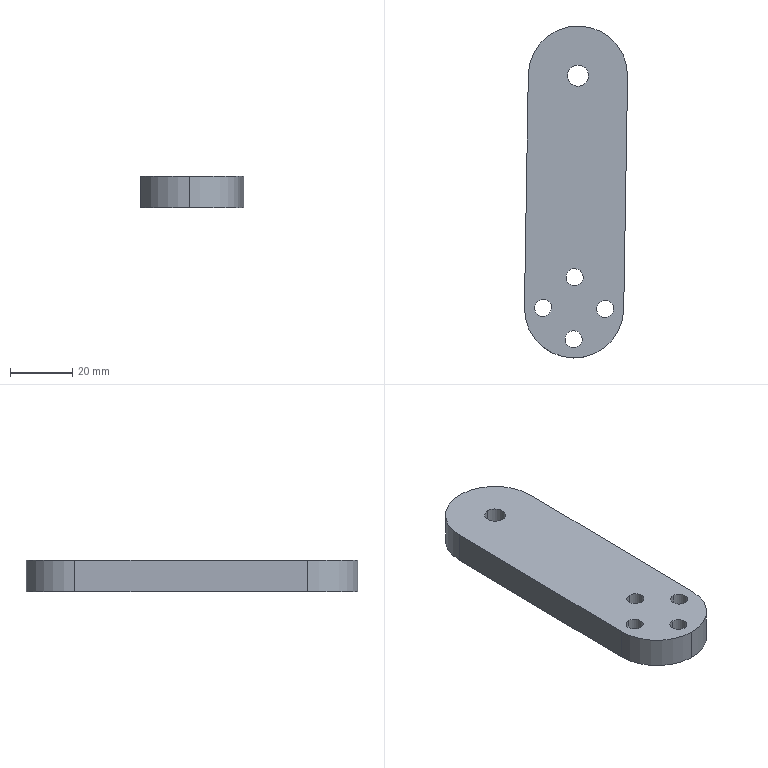Component | SolidWorks | 75-02-16StirringConnectingRod-1 | 1 solid | 29 faces | box 33.24 x 106.99 x 10 mm | volume 29480 mm3 | cylinder 21 | plane 8 | commonest cylinder face diameters 10 x8 5.5 x8 32 x3 6.8 x2 | material A3 Steel
build123d program:
from build123d import *

# Parameters (mm, degrees)
BOSS_EXTRUDE1_DEPTH                                = 5
HOLE_SIZE_ACCORDING_TO_TYPE_OF_HEXAGON_D           = 5.5
HOLE_SIZE_ACCORDING_TO_TYPE_OF_HEXAGON_CBORE_D     = 10
HOLE_SIZE_ACCORDING_TO_TYPE_OF_HEXAGON_CBORE_DEPTH = 5.7
M8_TAPPED_HOLE1_D                                  = 6.8


with BuildPart() as part:
    # Sketch1 → Boss-Extrude1 (new, symmetric)
    with BuildSketch(Plane.XY):
        with BuildLine():
            Line((-37.5, 16), (37.5, 16))
            ThreePointArc((37.5, 16), (53.5, 0), (37.5, -16))
            Line((37.5, -16), (-37.5, -16))
            ThreePointArc((-37.5, -16), (-53.5, 0), (-37.5, 16))
        make_face()
    extrude(amount=BOSS_EXTRUDE1_DEPTH, both=True)

    # Hole Size _according to_ Type of Hexagon (through all)
    with Locations(Plane(origin=(-37.5, 10, 5), x_dir=(1, 0, 0), z_dir=(0, 0, 1))):
        with Locations((0, 0), (10, -10), (-10, -10), (0, -20)):
            CounterBoreHole(HOLE_SIZE_ACCORDING_TO_TYPE_OF_HEXAGON_D / 2, HOLE_SIZE_ACCORDING_TO_TYPE_OF_HEXAGON_CBORE_D / 2, HOLE_SIZE_ACCORDING_TO_TYPE_OF_HEXAGON_CBORE_DEPTH)

    # M8 Tapped Hole1 (through all)
    with Locations(Plane(origin=(37.5, 0, 5), x_dir=(1, 0, 0), z_dir=(0, 0, 1))):
        with Locations((0, 0)):
            Hole(M8_TAPPED_HOLE1_D / 2)


solid = part.part

# Placed as in the assembly
solid = solid.moved(Location((-17.178, 49.362, 71.25), (-180, 0, -89.049)))
STEP:
#1=COLOUR_RGB('',0.7922,0.8196,0.9333);
#2=FILL_AREA_STYLE_COLOUR('',#1);
#3=FILL_AREA_STYLE('',(#2));
#4=SURFACE_STYLE_FILL_AREA(#3);
#5=SURFACE_SIDE_STYLE('',(#4));
#6=SURFACE_STYLE_USAGE(.BOTH.,#5);
#7=PRESENTATION_STYLE_ASSIGNMENT((#6));
#8=CARTESIAN_POINT('',(-0.654,3.286,3.002));
#9=VERTEX_POINT('',#8);
#10=CARTESIAN_POINT('',(-0.6496,3.553,3.002));
#11=VERTEX_POINT('',#10);
#12=CARTESIAN_POINT('',(-0.6518,3.42,3.002));
#13=DIRECTION('',(0.,0.,-1.));
#14=DIRECTION('',(0.0166,0.9999,0.));
#15=AXIS2_PLACEMENT_3D('',#12,#13,#14);
#16=CIRCLE('',#15,0.1339);
#17=EDGE_CURVE('',#9,#11,#16,.T.);
#18=ORIENTED_EDGE('',*,*,#17,.F.);
#19=CARTESIAN_POINT('',(-0.654,3.286,2.608));
#20=VERTEX_POINT('',#19);
#21=CARTESIAN_POINT('',(-0.654,3.286,2.608));
#22=DIRECTION('',(0.,0.,-1.));
#23=VECTOR('',#22,39.37);
#24=LINE('',#21,#23);
#25=EDGE_CURVE('',#9,#20,#24,.T.);
#26=ORIENTED_EDGE('',*,*,#25,.T.);
#27=CARTESIAN_POINT('',(-0.6496,3.553,2.608));
#28=VERTEX_POINT('',#27);
#29=CARTESIAN_POINT('',(-0.6518,3.42,2.608));
#30=DIRECTION('',(0.,0.,-1.));
#31=DIRECTION('',(0.0166,0.9999,0.));
#32=AXIS2_PLACEMENT_3D('',#29,#30,#31);
#33=CIRCLE('',#32,0.1339);
#34=EDGE_CURVE('',#20,#28,#33,.T.);
#35=ORIENTED_EDGE('',*,*,#34,.T.);
#36=CARTESIAN_POINT('',(-0.6496,3.553,2.608));
#37=DIRECTION('',(0.,0.,-1.));
#38=VECTOR('',#37,39.37);
#39=LINE('',#36,#38);
#40=EDGE_CURVE('',#11,#28,#39,.T.);
#41=ORIENTED_EDGE('',*,*,#40,.F.);
#42=EDGE_LOOP('',(#18,#26,#35,#41));
#43=FACE_OUTER_BOUND('',#42,.T.);
#44=CARTESIAN_POINT('',(-0.6518,3.42,2.608));
#45=DIRECTION('',(0.,0.,-1.));
#46=DIRECTION('',(0.0166,0.9999,0.));
#47=AXIS2_PLACEMENT_3D('',#44,#45,#46);
#48=CYLINDRICAL_SURFACE('',#47,0.1339);
#49=ADVANCED_FACE('',(#43),#48,.F.);
#50=CARTESIAN_POINT('',(-0.3104,0.2638,2.833));
#51=VERTEX_POINT('',#50);
#52=CARTESIAN_POINT('',(-0.3039,0.6575,2.833));
#53=VERTEX_POINT('',#52);
#54=CARTESIAN_POINT('',(-0.3072,0.4607,2.833));
#55=DIRECTION('',(0.,0.,-1.));
#56=DIRECTION('',(0.0166,0.9999,0.));
#57=AXIS2_PLACEMENT_3D('',#54,#55,#56);
#58=CIRCLE('',#57,0.1969);
#59=EDGE_CURVE('',#51,#53,#58,.T.);
#60=ORIENTED_EDGE('',*,*,#59,.F.);
#61=CARTESIAN_POINT('',(-0.3104,0.2638,2.608));
#62=VERTEX_POINT('',#61);
#63=CARTESIAN_POINT('',(-0.3104,0.2638,2.608));
#64=DIRECTION('',(0.,0.,-1.));
#65=VECTOR('',#64,39.37);
#66=LINE('',#63,#65);
#67=EDGE_CURVE('',#51,#62,#66,.T.);
#68=ORIENTED_EDGE('',*,*,#67,.T.);
#69=CARTESIAN_POINT('',(-0.3039,0.6575,2.608));
#70=VERTEX_POINT('',#69);
#71=CARTESIAN_POINT('',(-0.3072,0.4607,2.608));
#72=DIRECTION('',(0.,0.,-1.));
#73=DIRECTION('',(0.0166,0.9999,0.));
#74=AXIS2_PLACEMENT_3D('',#71,#72,#73);
#75=CIRCLE('',#74,0.1969);
#76=EDGE_CURVE('',#62,#70,#75,.T.);
#77=ORIENTED_EDGE('',*,*,#76,.T.);
#78=CARTESIAN_POINT('',(-0.3039,0.6575,2.608));
#79=DIRECTION('',(0.,0.,-1.));
#80=VECTOR('',#79,39.37);
#81=LINE('',#78,#80);
#82=EDGE_CURVE('',#53,#70,#81,.T.);
#83=ORIENTED_EDGE('',*,*,#82,.F.);
#84=EDGE_LOOP('',(#60,#68,#77,#83));
#85=FACE_OUTER_BOUND('',#84,.T.);
#86=CARTESIAN_POINT('',(-0.3072,0.4607,2.608));
#87=DIRECTION('',(0.,0.,-1.));
#88=DIRECTION('',(0.0166,0.9999,0.));
#89=AXIS2_PLACEMENT_3D('',#86,#87,#88);
#90=CYLINDRICAL_SURFACE('',#89,0.1969);
#91=ADVANCED_FACE('',(#85),#90,.F.);
#92=CARTESIAN_POINT('',(-0.309,0.3524,3.002));
#93=VERTEX_POINT('',#92);
#94=CARTESIAN_POINT('',(-0.3054,0.5689,3.002));
#95=VERTEX_POINT('',#94);
#96=CARTESIAN_POINT('',(-0.3072,0.4607,3.002));
#97=DIRECTION('',(0.,0.,-1.));
#98=DIRECTION('',(0.0166,0.9999,0.));
#99=AXIS2_PLACEMENT_3D('',#96,#97,#98);
#100=CIRCLE('',#99,0.1083);
#101=EDGE_CURVE('',#93,#95,#100,.T.);
#102=ORIENTED_EDGE('',*,*,#101,.F.);
#103=CARTESIAN_POINT('',(-0.309,0.3524,2.833));
#104=VERTEX_POINT('',#103);
#105=CARTESIAN_POINT('',(-0.309,0.3524,2.608));
#106=DIRECTION('',(0.,0.,-1.));
#107=VECTOR('',#106,39.37);
#108=LINE('',#105,#107);
#109=EDGE_CURVE('',#93,#104,#108,.T.);
#110=ORIENTED_EDGE('',*,*,#109,.T.);
#111=CARTESIAN_POINT('',(-0.3054,0.5689,2.833));
#112=VERTEX_POINT('',#111);
#113=CARTESIAN_POINT('',(-0.3072,0.4607,2.833));
#114=DIRECTION('',(0.,0.,-1.));
#115=DIRECTION('',(0.0166,0.9999,0.));
#116=AXIS2_PLACEMENT_3D('',#113,#114,#115);
#117=CIRCLE('',#116,0.1083);
#118=EDGE_CURVE('',#104,#112,#117,.T.);
#119=ORIENTED_EDGE('',*,*,#118,.T.);
#120=CARTESIAN_POINT('',(-0.3054,0.5689,2.608));
#121=DIRECTION('',(0.,0.,-1.));
#122=VECTOR('',#121,39.37);
#123=LINE('',#120,#122);
#124=EDGE_CURVE('',#95,#112,#123,.T.);
#125=ORIENTED_EDGE('',*,*,#124,.F.);
#126=EDGE_LOOP('',(#102,#110,#119,#125));
#127=FACE_OUTER_BOUND('',#126,.T.);
#128=CARTESIAN_POINT('',(-0.3072,0.4607,2.608));
#129=DIRECTION('',(0.,0.,-1.));
#130=DIRECTION('',(0.0166,0.9999,0.));
#131=AXIS2_PLACEMENT_3D('',#128,#129,#130);
#132=CYLINDRICAL_SURFACE('',#131,0.1083);
#133=ADVANCED_FACE('',(#127),#132,.F.);
#134=CARTESIAN_POINT('',(-0.6975,0.664,2.833));
#135=VERTEX_POINT('',#134);
#136=CARTESIAN_POINT('',(-0.691,1.058,2.833));
#137=VERTEX_POINT('',#136);
#138=CARTESIAN_POINT('',(-0.6943,0.8608,2.833));
#139=DIRECTION('',(0.,0.,-1.));
#140=DIRECTION('',(0.0166,0.9999,0.));
#141=AXIS2_PLACEMENT_3D('',#138,#139,#140);
#142=CIRCLE('',#141,0.1969);
#143=EDGE_CURVE('',#135,#137,#142,.T.);
#144=ORIENTED_EDGE('',*,*,#143,.F.);
#145=CARTESIAN_POINT('',(-0.6975,0.664,2.608));
#146=VERTEX_POINT('',#145);
#147=CARTESIAN_POINT('',(-0.6975,0.664,2.608));
#148=DIRECTION('',(0.,0.,-1.));
#149=VECTOR('',#148,39.37);
#150=LINE('',#147,#149);
#151=EDGE_CURVE('',#135,#146,#150,.T.);
#152=ORIENTED_EDGE('',*,*,#151,.T.);
#153=CARTESIAN_POINT('',(-0.691,1.058,2.608));
#154=VERTEX_POINT('',#153);
#155=CARTESIAN_POINT('',(-0.6943,0.8608,2.608));
#156=DIRECTION('',(0.,0.,-1.));
#157=DIRECTION('',(0.0166,0.9999,0.));
#158=AXIS2_PLACEMENT_3D('',#155,#156,#157);
#159=CIRCLE('',#158,0.1969);
#160=EDGE_CURVE('',#146,#154,#159,.T.);
#161=ORIENTED_EDGE('',*,*,#160,.T.);
#162=CARTESIAN_POINT('',(-0.691,1.058,2.608));
#163=DIRECTION('',(0.,0.,-1.));
#164=VECTOR('',#163,39.37);
#165=LINE('',#162,#164);
#166=EDGE_CURVE('',#137,#154,#165,.T.);
#167=ORIENTED_EDGE('',*,*,#166,.F.);
#168=EDGE_LOOP('',(#144,#152,#161,#167));
#169=FACE_OUTER_BOUND('',#168,.T.);
#170=CARTESIAN_POINT('',(-0.6943,0.8608,2.608));
#171=DIRECTION('',(0.,0.,-1.));
#172=DIRECTION('',(0.0166,0.9999,0.));
#173=AXIS2_PLACEMENT_3D('',#170,#171,#172);
#174=CYLINDRICAL_SURFACE('',#173,0.1969);
#175=ADVANCED_FACE('',(#169),#174,.F.);
#176=CARTESIAN_POINT('',(-0.6961,0.7526,3.002));
#177=VERTEX_POINT('',#176);
#178=CARTESIAN_POINT('',(-0.6925,0.9691,3.002));
#179=VERTEX_POINT('',#178);
#180=CARTESIAN_POINT('',(-0.6943,0.8608,3.002));
#181=DIRECTION('',(0.,0.,-1.));
#182=DIRECTION('',(0.0166,0.9999,0.));
#183=AXIS2_PLACEMENT_3D('',#180,#181,#182);
#184=CIRCLE('',#183,0.1083);
#185=EDGE_CURVE('',#177,#179,#184,.T.);
#186=ORIENTED_EDGE('',*,*,#185,.F.);
#187=CARTESIAN_POINT('',(-0.6961,0.7526,2.833));
#188=VERTEX_POINT('',#187);
#189=CARTESIAN_POINT('',(-0.6961,0.7526,2.608));
#190=DIRECTION('',(0.,0.,-1.));
#191=VECTOR('',#190,39.37);
#192=LINE('',#189,#191);
#193=EDGE_CURVE('',#177,#188,#192,.T.);
#194=ORIENTED_EDGE('',*,*,#193,.T.);
#195=CARTESIAN_POINT('',(-0.6925,0.9691,2.833));
#196=VERTEX_POINT('',#195);
#197=CARTESIAN_POINT('',(-0.6943,0.8608,2.833));
#198=DIRECTION('',(0.,0.,-1.));
#199=DIRECTION('',(0.0166,0.9999,0.));
#200=AXIS2_PLACEMENT_3D('',#197,#198,#199);
#201=CIRCLE('',#200,0.1083);
#202=EDGE_CURVE('',#188,#196,#201,.T.);
#203=ORIENTED_EDGE('',*,*,#202,.T.);
#204=CARTESIAN_POINT('',(-0.6925,0.9691,2.608));
#205=DIRECTION('',(0.,0.,-1.));
#206=VECTOR('',#205,39.37);
#207=LINE('',#204,#206);
#208=EDGE_CURVE('',#179,#196,#207,.T.);
#209=ORIENTED_EDGE('',*,*,#208,.F.);
#210=EDGE_LOOP('',(#186,#194,#203,#209));
#211=FACE_OUTER_BOUND('',#210,.T.);
#212=CARTESIAN_POINT('',(-0.6943,0.8608,2.608));
#213=DIRECTION('',(0.,0.,-1.));
#214=DIRECTION('',(0.0166,0.9999,0.));
#215=AXIS2_PLACEMENT_3D('',#212,#213,#214);
#216=CYLINDRICAL_SURFACE('',#215,0.1083);
#217=ADVANCED_FACE('',(#211),#216,.F.);
#218=CARTESIAN_POINT('',(-0.7106,-0.1233,2.833));
#219=VERTEX_POINT('',#218);
#220=CARTESIAN_POINT('',(-0.7041,0.2704,2.833));
#221=VERTEX_POINT('',#220);
#222=CARTESIAN_POINT('',(-0.7073,0.07355,2.833));
#223=DIRECTION('',(0.,0.,-1.));
#224=DIRECTION('',(0.0166,0.9999,0.));
#225=AXIS2_PLACEMENT_3D('',#222,#223,#224);
#226=CIRCLE('',#225,0.1969);
#227=EDGE_CURVE('',#219,#221,#226,.T.);
#228=ORIENTED_EDGE('',*,*,#227,.F.);
#229=CARTESIAN_POINT('',(-0.7106,-0.1233,2.608));
#230=VERTEX_POINT('',#229);
#231=CARTESIAN_POINT('',(-0.7106,-0.1233,2.608));
#232=DIRECTION('',(0.,0.,-1.));
#233=VECTOR('',#232,39.37);
#234=LINE('',#231,#233);
#235=EDGE_CURVE('',#219,#230,#234,.T.);
#236=ORIENTED_EDGE('',*,*,#235,.T.);
#237=CARTESIAN_POINT('',(-0.7041,0.2704,2.608));
#238=VERTEX_POINT('',#237);
#239=CARTESIAN_POINT('',(-0.7073,0.07355,2.608));
#240=DIRECTION('',(0.,0.,-1.));
#241=DIRECTION('',(0.0166,0.9999,0.));
#242=AXIS2_PLACEMENT_3D('',#239,#240,#241);
#243=CIRCLE('',#242,0.1969);
#244=EDGE_CURVE('',#230,#238,#243,.T.);
#245=ORIENTED_EDGE('',*,*,#244,.T.);
#246=CARTESIAN_POINT('',(-0.7041,0.2704,2.608));
#247=DIRECTION('',(0.,0.,-1.));
#248=VECTOR('',#247,39.37);
#249=LINE('',#246,#248);
#250=EDGE_CURVE('',#221,#238,#249,.T.);
#251=ORIENTED_EDGE('',*,*,#250,.F.);
#252=EDGE_LOOP('',(#228,#236,#245,#251));
#253=FACE_OUTER_BOUND('',#252,.T.);
#254=CARTESIAN_POINT('',(-0.7073,0.07355,2.608));
#255=DIRECTION('',(0.,0.,-1.));
#256=DIRECTION('',(0.0166,0.9999,0.));
#257=AXIS2_PLACEMENT_3D('',#254,#255,#256);
#258=CYLINDRICAL_SURFACE('',#257,0.1969);
#259=ADVANCED_FACE('',(#253),#258,.F.);
#260=CARTESIAN_POINT('',(-0.7091,-0.0347,3.002));
#261=VERTEX_POINT('',#260);
#262=CARTESIAN_POINT('',(-0.7055,0.1818,3.002));
#263=VERTEX_POINT('',#262);
#264=CARTESIAN_POINT('',(-0.7073,0.07355,3.002));
#265=DIRECTION('',(0.,0.,-1.));
#266=DIRECTION('',(0.0166,0.9999,0.));
#267=AXIS2_PLACEMENT_3D('',#264,#265,#266);
#268=CIRCLE('',#267,0.1083);
#269=EDGE_CURVE('',#261,#263,#268,.T.);
#270=ORIENTED_EDGE('',*,*,#269,.F.);
#271=CARTESIAN_POINT('',(-0.7091,-0.0347,2.833));
#272=VERTEX_POINT('',#271);
#273=CARTESIAN_POINT('',(-0.7091,-0.0347,2.608));
#274=DIRECTION('',(0.,0.,-1.));
#275=VECTOR('',#274,39.37);
#276=LINE('',#273,#275);
#277=EDGE_CURVE('',#261,#272,#276,.T.);
#278=ORIENTED_EDGE('',*,*,#277,.T.);
#279=CARTESIAN_POINT('',(-0.7055,0.1818,2.833));
#280=VERTEX_POINT('',#279);
#281=CARTESIAN_POINT('',(-0.7073,0.07355,2.833));
#282=DIRECTION('',(0.,0.,-1.));
#283=DIRECTION('',(0.0166,0.9999,0.));
#284=AXIS2_PLACEMENT_3D('',#281,#282,#283);
#285=CIRCLE('',#284,0.1083);
#286=EDGE_CURVE('',#272,#280,#285,.T.);
#287=ORIENTED_EDGE('',*,*,#286,.T.);
#288=CARTESIAN_POINT('',(-0.7055,0.1818,2.608));
#289=DIRECTION('',(0.,0.,-1.));
#290=VECTOR('',#289,39.37);
#291=LINE('',#288,#290);
#292=EDGE_CURVE('',#263,#280,#291,.T.);
#293=ORIENTED_EDGE('',*,*,#292,.F.);
#294=EDGE_LOOP('',(#270,#278,#287,#293));
#295=FACE_OUTER_BOUND('',#294,.T.);
#296=CARTESIAN_POINT('',(-0.7073,0.07355,2.608));
#297=DIRECTION('',(0.,0.,-1.));
#298=DIRECTION('',(0.0166,0.9999,0.));
#299=AXIS2_PLACEMENT_3D('',#296,#297,#298);
#300=CYLINDRICAL_SURFACE('',#299,0.1083);
#301=ADVANCED_FACE('',(#295),#300,.F.);
#302=CARTESIAN_POINT('',(-1.098,0.2769,2.833));
#303=VERTEX_POINT('',#302);
#304=CARTESIAN_POINT('',(-1.091,0.6706,2.833));
#305=VERTEX_POINT('',#304);
#306=CARTESIAN_POINT('',(-1.094,0.4737,2.833));
#307=DIRECTION('',(0.,0.,-1.));
#308=DIRECTION('',(0.0166,0.9999,0.));
#309=AXIS2_PLACEMENT_3D('',#306,#307,#308);
#310=CIRCLE('',#309,0.1969);
#311=EDGE_CURVE('',#303,#305,#310,.T.);
#312=ORIENTED_EDGE('',*,*,#311,.F.);
#313=CARTESIAN_POINT('',(-1.098,0.2769,2.608));
#314=VERTEX_POINT('',#313);
#315=CARTESIAN_POINT('',(-1.098,0.2769,2.608));
#316=DIRECTION('',(0.,0.,-1.));
#317=VECTOR('',#316,39.37);
#318=LINE('',#315,#317);
#319=EDGE_CURVE('',#303,#314,#318,.T.);
#320=ORIENTED_EDGE('',*,*,#319,.T.);
#321=CARTESIAN_POINT('',(-1.091,0.6706,2.608));
#322=VERTEX_POINT('',#321);
#323=CARTESIAN_POINT('',(-1.094,0.4737,2.608));
#324=DIRECTION('',(0.,0.,-1.));
#325=DIRECTION('',(0.0166,0.9999,0.));
#326=AXIS2_PLACEMENT_3D('',#323,#324,#325);
#327=CIRCLE('',#326,0.1969);
#328=EDGE_CURVE('',#314,#322,#327,.T.);
#329=ORIENTED_EDGE('',*,*,#328,.T.);
#330=CARTESIAN_POINT('',(-1.091,0.6706,2.608));
#331=DIRECTION('',(0.,0.,-1.));
#332=VECTOR('',#331,39.37);
#333=LINE('',#330,#332);
#334=EDGE_CURVE('',#305,#322,#333,.T.);
#335=ORIENTED_EDGE('',*,*,#334,.F.);
#336=EDGE_LOOP('',(#312,#320,#329,#335));
#337=FACE_OUTER_BOUND('',#336,.T.);
#338=CARTESIAN_POINT('',(-1.094,0.4737,2.608));
#339=DIRECTION('',(0.,0.,-1.));
#340=DIRECTION('',(0.0166,0.9999,0.));
#341=AXIS2_PLACEMENT_3D('',#338,#339,#340);
#342=CYLINDRICAL_SURFACE('',#341,0.1969);
#343=ADVANCED_FACE('',(#337),#342,.F.);
#344=CARTESIAN_POINT('',(-1.096,0.3655,3.002));
#345=VERTEX_POINT('',#344);
#346=CARTESIAN_POINT('',(-1.093,0.582,3.002));
#347=VERTEX_POINT('',#346);
#348=CARTESIAN_POINT('',(-1.094,0.4737,3.002));
#349=DIRECTION('',(0.,0.,-1.));
#350=DIRECTION('',(0.0166,0.9999,0.));
#351=AXIS2_PLACEMENT_3D('',#348,#349,#350);
#352=CIRCLE('',#351,0.1083);
#353=EDGE_CURVE('',#345,#347,#352,.T.);
#354=ORIENTED_EDGE('',*,*,#353,.F.);
#355=CARTESIAN_POINT('',(-1.096,0.3655,2.833));
#356=VERTEX_POINT('',#355);
#357=CARTESIAN_POINT('',(-1.096,0.3655,2.608));
#358=DIRECTION('',(0.,0.,-1.));
#359=VECTOR('',#358,39.37);
#360=LINE('',#357,#359);
#361=EDGE_CURVE('',#345,#356,#360,.T.);
#362=ORIENTED_EDGE('',*,*,#361,.T.);
#363=CARTESIAN_POINT('',(-1.093,0.582,2.833));
#364=VERTEX_POINT('',#363);
#365=CARTESIAN_POINT('',(-1.094,0.4737,2.833));
#366=DIRECTION('',(0.,0.,-1.));
#367=DIRECTION('',(0.0166,0.9999,0.));
#368=AXIS2_PLACEMENT_3D('',#365,#366,#367);
#369=CIRCLE('',#368,0.1083);
#370=EDGE_CURVE('',#356,#364,#369,.T.);
#371=ORIENTED_EDGE('',*,*,#370,.T.);
#372=CARTESIAN_POINT('',(-1.093,0.582,2.608));
#373=DIRECTION('',(0.,0.,-1.));
#374=VECTOR('',#373,39.37);
#375=LINE('',#372,#374);
#376=EDGE_CURVE('',#347,#364,#375,.T.);
#377=ORIENTED_EDGE('',*,*,#376,.F.);
#378=EDGE_LOOP('',(#354,#362,#371,#377));
#379=FACE_OUTER_BOUND('',#378,.T.);
#380=CARTESIAN_POINT('',(-1.094,0.4737,2.608));
#381=DIRECTION('',(0.,0.,-1.));
#382=DIRECTION('',(0.0166,0.9999,0.));
#383=AXIS2_PLACEMENT_3D('',#380,#381,#382);
#384=CYLINDRICAL_SURFACE('',#383,0.1083);
#385=ADVANCED_FACE('',(#379),#384,.F.);
#386=CARTESIAN_POINT('',(-0.7113,-0.1626,2.608));
#387=VERTEX_POINT('',#386);
#388=CARTESIAN_POINT('',(-1.331,0.4777,2.608));
#389=VERTEX_POINT('',#388);
#390=CARTESIAN_POINT('',(-0.7008,0.4672,2.608));
#391=DIRECTION('',(0.,0.,-1.));
#392=DIRECTION('',(0.0166,0.9999,0.));
#393=AXIS2_PLACEMENT_3D('',#390,#391,#392);
#394=CIRCLE('',#393,0.6299);
#395=EDGE_CURVE('',#387,#389,#394,.T.);
#396=ORIENTED_EDGE('',*,*,#395,.F.);
#397=CARTESIAN_POINT('',(-0.7113,-0.1626,3.002));
#398=VERTEX_POINT('',#397);
#399=CARTESIAN_POINT('',(-0.7113,-0.1626,2.608));
#400=DIRECTION('',(-0.,-0.,1.));
#401=VECTOR('',#400,39.37);
#402=LINE('',#399,#401);
#403=EDGE_CURVE('',#387,#398,#402,.T.);
#404=ORIENTED_EDGE('',*,*,#403,.T.);
#405=CARTESIAN_POINT('',(-1.331,0.4777,3.002));
#406=VERTEX_POINT('',#405);
#407=CARTESIAN_POINT('',(-0.7008,0.4672,3.002));
#408=DIRECTION('',(0.,0.,-1.));
#409=DIRECTION('',(0.0166,0.9999,0.));
#410=AXIS2_PLACEMENT_3D('',#407,#408,#409);
#411=CIRCLE('',#410,0.6299);
#412=EDGE_CURVE('',#398,#406,#411,.T.);
#413=ORIENTED_EDGE('',*,*,#412,.T.);
#414=CARTESIAN_POINT('',(-1.331,0.4777,2.608));
#415=DIRECTION('',(-0.,-0.,1.));
#416=VECTOR('',#415,39.37);
#417=LINE('',#414,#416);
#418=EDGE_CURVE('',#389,#406,#417,.T.);
#419=ORIENTED_EDGE('',*,*,#418,.F.);
#420=EDGE_LOOP('',(#396,#404,#413,#419));
#421=FACE_OUTER_BOUND('',#420,.T.);
#422=CARTESIAN_POINT('',(-0.7008,0.4672,2.608));
#423=DIRECTION('',(-0.,-0.,1.));
#424=DIRECTION('',(-0.0166,-0.9999,0.));
#425=AXIS2_PLACEMENT_3D('',#422,#423,#424);
#426=CYLINDRICAL_SURFACE('',#425,0.6299);
#427=ADVANCED_FACE('',(#421),#426,.T.);
#428=ORIENTED_EDGE('',*,*,#403,.F.);
#429=CARTESIAN_POINT('',(-0.07097,0.4567,2.608));
#430=VERTEX_POINT('',#429);
#431=CARTESIAN_POINT('',(-0.7008,0.4672,2.608));
#432=DIRECTION('',(0.,0.,-1.));
#433=DIRECTION('',(0.0166,0.9999,0.));
#434=AXIS2_PLACEMENT_3D('',#431,#432,#433);
#435=CIRCLE('',#434,0.6299);
#436=EDGE_CURVE('',#430,#387,#435,.T.);
#437=ORIENTED_EDGE('',*,*,#436,.F.);
#438=CARTESIAN_POINT('',(-0.07097,0.4567,3.002));
#439=VERTEX_POINT('',#438);
#440=CARTESIAN_POINT('',(-0.07097,0.4567,2.608));
#441=DIRECTION('',(-0.,-0.,1.));
#442=VECTOR('',#441,39.37);
#443=LINE('',#440,#442);
#444=EDGE_CURVE('',#430,#439,#443,.T.);
#445=ORIENTED_EDGE('',*,*,#444,.T.);
#446=CARTESIAN_POINT('',(-0.7008,0.4672,3.002));
#447=DIRECTION('',(0.,0.,-1.));
#448=DIRECTION('',(0.0166,0.9999,0.));
#449=AXIS2_PLACEMENT_3D('',#446,#447,#448);
#450=CIRCLE('',#449,0.6299);
#451=EDGE_CURVE('',#439,#398,#450,.T.);
#452=ORIENTED_EDGE('',*,*,#451,.T.);
#453=EDGE_LOOP('',(#428,#437,#445,#452));
#454=FACE_OUTER_BOUND('',#453,.T.);
#455=CARTESIAN_POINT('',(-0.7008,0.4672,2.608));
#456=DIRECTION('',(-0.,-0.,1.));
#457=DIRECTION('',(-0.0166,-0.9999,0.));
#458=AXIS2_PLACEMENT_3D('',#455,#456,#457);
#459=CYLINDRICAL_SURFACE('',#458,0.6299);
#460=ADVANCED_FACE('',(#454),#459,.T.);
#461=CARTESIAN_POINT('',(-1.282,3.43,3.002));
#462=VERTEX_POINT('',#461);
#463=CARTESIAN_POINT('',(-1.331,0.4777,3.002));
#464=DIRECTION('',(0.0166,0.9999,0.));
#465=VECTOR('',#464,39.37);
#466=LINE('',#463,#465);
#467=EDGE_CURVE('',#406,#462,#466,.T.);
#468=ORIENTED_EDGE('',*,*,#467,.T.);
#469=CARTESIAN_POINT('',(-1.282,3.43,2.608));
#470=VERTEX_POINT('',#469);
#471=CARTESIAN_POINT('',(-1.282,3.43,2.608));
#472=DIRECTION('',(-0.,-0.,1.));
#473=VECTOR('',#472,39.37);
#474=LINE('',#471,#473);
#475=EDGE_CURVE('',#470,#462,#474,.T.);
#476=ORIENTED_EDGE('',*,*,#475,.F.);
#477=CARTESIAN_POINT('',(-1.331,0.4777,2.608));
#478=DIRECTION('',(0.0166,0.9999,0.));
#479=VECTOR('',#478,39.37);
#480=LINE('',#477,#479);
#481=EDGE_CURVE('',#389,#470,#480,.T.);
#482=ORIENTED_EDGE('',*,*,#481,.F.);
#483=ORIENTED_EDGE('',*,*,#418,.T.);
#484=EDGE_LOOP('',(#468,#476,#482,#483));
#485=FACE_OUTER_BOUND('',#484,.T.);
#486=CARTESIAN_POINT('',(-1.331,0.4777,2.608));
#487=DIRECTION('',(0.9999,-0.0166,0.));
#488=DIRECTION('',(0.,0.,-1.));
#489=AXIS2_PLACEMENT_3D('',#486,#487,#488);
#490=PLANE('',#489);
#491=ADVANCED_FACE('',(#485),#490,.F.);
#492=CARTESIAN_POINT('',(-0.02196,3.409,3.002));
#493=VERTEX_POINT('',#492);
#494=CARTESIAN_POINT('',(-0.6518,3.42,3.002));
#495=DIRECTION('',(0.,0.,-1.));
#496=DIRECTION('',(0.0166,0.9999,0.));
#497=AXIS2_PLACEMENT_3D('',#494,#495,#496);
#498=CIRCLE('',#497,0.6299);
#499=EDGE_CURVE('',#462,#493,#498,.T.);
#500=ORIENTED_EDGE('',*,*,#499,.T.);
#501=CARTESIAN_POINT('',(-0.02196,3.409,2.608));
#502=VERTEX_POINT('',#501);
#503=CARTESIAN_POINT('',(-0.02196,3.409,2.608));
#504=DIRECTION('',(-0.,-0.,1.));
#505=VECTOR('',#504,39.37);
#506=LINE('',#503,#505);
#507=EDGE_CURVE('',#502,#493,#506,.T.);
#508=ORIENTED_EDGE('',*,*,#507,.F.);
#509=CARTESIAN_POINT('',(-0.6518,3.42,2.608));
#510=DIRECTION('',(0.,0.,-1.));
#511=DIRECTION('',(0.0166,0.9999,0.));
#512=AXIS2_PLACEMENT_3D('',#509,#510,#511);
#513=CIRCLE('',#512,0.6299);
#514=EDGE_CURVE('',#470,#502,#513,.T.);
#515=ORIENTED_EDGE('',*,*,#514,.F.);
#516=ORIENTED_EDGE('',*,*,#475,.T.);
#517=EDGE_LOOP('',(#500,#508,#515,#516));
#518=FACE_OUTER_BOUND('',#517,.T.);
#519=CARTESIAN_POINT('',(-0.6518,3.42,2.608));
#520=DIRECTION('',(-0.,-0.,1.));
#521=DIRECTION('',(-0.0166,-0.9999,0.));
#522=AXIS2_PLACEMENT_3D('',#519,#520,#521);
#523=CYLINDRICAL_SURFACE('',#522,0.6299);
#524=ADVANCED_FACE('',(#518),#523,.T.);
#525=CARTESIAN_POINT('',(-0.07097,0.4567,3.002));
#526=DIRECTION('',(-0.0166,-0.9999,-0.));
#527=VECTOR('',#526,39.37);
#528=LINE('',#525,#527);
#529=EDGE_CURVE('',#493,#439,#528,.T.);
#530=ORIENTED_EDGE('',*,*,#529,.T.);
#531=ORIENTED_EDGE('',*,*,#444,.F.);
#532=CARTESIAN_POINT('',(-0.07097,0.4567,2.608));
#533=DIRECTION('',(-0.0166,-0.9999,-0.));
#534=VECTOR('',#533,39.37);
#535=LINE('',#532,#534);
#536=EDGE_CURVE('',#502,#430,#535,.T.);
#537=ORIENTED_EDGE('',*,*,#536,.F.);
#538=ORIENTED_EDGE('',*,*,#507,.T.);
#539=EDGE_LOOP('',(#530,#531,#537,#538));
#540=FACE_OUTER_BOUND('',#539,.T.);
#541=CARTESIAN_POINT('',(-0.07097,0.4567,2.608));
#542=DIRECTION('',(-0.9999,0.0166,-0.));
#543=DIRECTION('',(-0.,-0.,1.));
#544=AXIS2_PLACEMENT_3D('',#541,#542,#543);
#545=PLANE('',#544);
#546=ADVANCED_FACE('',(#540),#545,.F.);
#547=CARTESIAN_POINT('',(-0.6518,3.42,2.608));
#548=DIRECTION('',(0.,0.,-1.));
#549=DIRECTION('',(0.0166,0.9999,0.));
#550=AXIS2_PLACEMENT_3D('',#547,#548,#549);
#551=CIRCLE('',#550,0.1339);
#552=EDGE_CURVE('',#28,#20,#551,.T.);
#553=ORIENTED_EDGE('',*,*,#552,.F.);
#554=ORIENTED_EDGE('',*,*,#34,.F.);
#555=EDGE_LOOP('',(#553,#554));
#556=FACE_BOUND('',#555,.T.);
#557=CARTESIAN_POINT('',(-0.3072,0.4607,2.608));
#558=DIRECTION('',(0.,0.,-1.));
#559=DIRECTION('',(0.0166,0.9999,0.));
#560=AXIS2_PLACEMENT_3D('',#557,#558,#559);
#561=CIRCLE('',#560,0.1969);
#562=EDGE_CURVE('',#70,#62,#561,.T.);
#563=ORIENTED_EDGE('',*,*,#562,.F.);
#564=ORIENTED_EDGE('',*,*,#76,.F.);
#565=EDGE_LOOP('',(#563,#564));
#566=FACE_BOUND('',#565,.T.);
#567=CARTESIAN_POINT('',(-0.6943,0.8608,2.608));
#568=DIRECTION('',(0.,0.,-1.));
#569=DIRECTION('',(0.0166,0.9999,0.));
#570=AXIS2_PLACEMENT_3D('',#567,#568,#569);
#571=CIRCLE('',#570,0.1969);
#572=EDGE_CURVE('',#154,#146,#571,.T.);
#573=ORIENTED_EDGE('',*,*,#572,.F.);
#574=ORIENTED_EDGE('',*,*,#160,.F.);
#575=EDGE_LOOP('',(#573,#574));
#576=FACE_BOUND('',#575,.T.);
#577=CARTESIAN_POINT('',(-0.7073,0.07355,2.608));
#578=DIRECTION('',(0.,0.,-1.));
#579=DIRECTION('',(0.0166,0.9999,0.));
#580=AXIS2_PLACEMENT_3D('',#577,#578,#579);
#581=CIRCLE('',#580,0.1969);
#582=EDGE_CURVE('',#238,#230,#581,.T.);
#583=ORIENTED_EDGE('',*,*,#582,.F.);
#584=ORIENTED_EDGE('',*,*,#244,.F.);
#585=EDGE_LOOP('',(#583,#584));
#586=FACE_BOUND('',#585,.T.);
#587=CARTESIAN_POINT('',(-1.094,0.4737,2.608));
#588=DIRECTION('',(0.,0.,-1.));
#589=DIRECTION('',(0.0166,0.9999,0.));
#590=AXIS2_PLACEMENT_3D('',#587,#588,#589);
#591=CIRCLE('',#590,0.1969);
#592=EDGE_CURVE('',#322,#314,#591,.T.);
#593=ORIENTED_EDGE('',*,*,#592,.F.);
#594=ORIENTED_EDGE('',*,*,#328,.F.);
#595=EDGE_LOOP('',(#593,#594));
#596=FACE_BOUND('',#595,.T.);
#597=ORIENTED_EDGE('',*,*,#436,.T.);
#598=ORIENTED_EDGE('',*,*,#395,.T.);
#599=ORIENTED_EDGE('',*,*,#481,.T.);
#600=ORIENTED_EDGE('',*,*,#514,.T.);
#601=ORIENTED_EDGE('',*,*,#536,.T.);
#602=EDGE_LOOP('',(#597,#598,#599,#600,#601));
#603=FACE_OUTER_BOUND('',#602,.T.);
#604=CARTESIAN_POINT('',(-0.7008,0.4672,2.608));
#605=DIRECTION('',(0.,0.,-1.));
#606=DIRECTION('',(0.0166,0.9999,0.));
#607=AXIS2_PLACEMENT_3D('',#604,#605,#606);
#608=PLANE('',#607);
#609=ADVANCED_FACE('',(#556,#566,#576,#586,#596,#603),#608,.T.);
#610=CARTESIAN_POINT('',(-0.6518,3.42,3.002));
#611=DIRECTION('',(0.,0.,-1.));
#612=DIRECTION('',(0.0166,0.9999,0.));
#613=AXIS2_PLACEMENT_3D('',#610,#611,#612);
#614=CIRCLE('',#613,0.1339);
#615=EDGE_CURVE('',#11,#9,#614,.T.);
#616=ORIENTED_EDGE('',*,*,#615,.T.);
#617=ORIENTED_EDGE('',*,*,#17,.T.);
#618=EDGE_LOOP('',(#616,#617));
#619=FACE_BOUND('',#618,.T.);
#620=CARTESIAN_POINT('',(-0.3072,0.4607,3.002));
#621=DIRECTION('',(0.,0.,-1.));
#622=DIRECTION('',(0.0166,0.9999,0.));
#623=AXIS2_PLACEMENT_3D('',#620,#621,#622);
#624=CIRCLE('',#623,0.1083);
#625=EDGE_CURVE('',#95,#93,#624,.T.);
#626=ORIENTED_EDGE('',*,*,#625,.T.);
#627=ORIENTED_EDGE('',*,*,#101,.T.);
#628=EDGE_LOOP('',(#626,#627));
#629=FACE_BOUND('',#628,.T.);
#630=CARTESIAN_POINT('',(-0.6943,0.8608,3.002));
#631=DIRECTION('',(0.,0.,-1.));
#632=DIRECTION('',(0.0166,0.9999,0.));
#633=AXIS2_PLACEMENT_3D('',#630,#631,#632);
#634=CIRCLE('',#633,0.1083);
#635=EDGE_CURVE('',#179,#177,#634,.T.);
#636=ORIENTED_EDGE('',*,*,#635,.T.);
#637=ORIENTED_EDGE('',*,*,#185,.T.);
#638=EDGE_LOOP('',(#636,#637));
#639=FACE_BOUND('',#638,.T.);
#640=CARTESIAN_POINT('',(-0.7073,0.07355,3.002));
#641=DIRECTION('',(0.,0.,-1.));
#642=DIRECTION('',(0.0166,0.9999,0.));
#643=AXIS2_PLACEMENT_3D('',#640,#641,#642);
#644=CIRCLE('',#643,0.1083);
#645=EDGE_CURVE('',#263,#261,#644,.T.);
#646=ORIENTED_EDGE('',*,*,#645,.T.);
#647=ORIENTED_EDGE('',*,*,#269,.T.);
#648=EDGE_LOOP('',(#646,#647));
#649=FACE_BOUND('',#648,.T.);
#650=CARTESIAN_POINT('',(-1.094,0.4737,3.002));
#651=DIRECTION('',(0.,0.,-1.));
#652=DIRECTION('',(0.0166,0.9999,0.));
#653=AXIS2_PLACEMENT_3D('',#650,#651,#652);
#654=CIRCLE('',#653,0.1083);
#655=EDGE_CURVE('',#347,#345,#654,.T.);
#656=ORIENTED_EDGE('',*,*,#655,.T.);
#657=ORIENTED_EDGE('',*,*,#353,.T.);
#658=EDGE_LOOP('',(#656,#657));
#659=FACE_BOUND('',#658,.T.);
#660=ORIENTED_EDGE('',*,*,#451,.F.);
#661=ORIENTED_EDGE('',*,*,#529,.F.);
#662=ORIENTED_EDGE('',*,*,#499,.F.);
#663=ORIENTED_EDGE('',*,*,#467,.F.);
#664=ORIENTED_EDGE('',*,*,#412,.F.);
#665=EDGE_LOOP('',(#660,#661,#662,#663,#664));
#666=FACE_OUTER_BOUND('',#665,.T.);
#667=CARTESIAN_POINT('',(-0.7008,0.4672,3.002));
#668=DIRECTION('',(0.,0.,-1.));
#669=DIRECTION('',(0.0166,0.9999,0.));
#670=AXIS2_PLACEMENT_3D('',#667,#668,#669);
#671=PLANE('',#670);
#672=ADVANCED_FACE('',(#619,#629,#639,#649,#659,#666),#671,.F.);
#673=ORIENTED_EDGE('',*,*,#361,.F.);
#674=ORIENTED_EDGE('',*,*,#655,.F.);
#675=ORIENTED_EDGE('',*,*,#376,.T.);
#676=CARTESIAN_POINT('',(-1.094,0.4737,2.833));
#677=DIRECTION('',(0.,0.,-1.));
#678=DIRECTION('',(0.0166,0.9999,0.));
#679=AXIS2_PLACEMENT_3D('',#676,#677,#678);
#680=CIRCLE('',#679,0.1083);
#681=EDGE_CURVE('',#364,#356,#680,.T.);
#682=ORIENTED_EDGE('',*,*,#681,.T.);
#683=EDGE_LOOP('',(#673,#674,#675,#682));
#684=FACE_OUTER_BOUND('',#683,.T.);
#685=CARTESIAN_POINT('',(-1.094,0.4737,2.608));
#686=DIRECTION('',(0.,0.,-1.));
#687=DIRECTION('',(0.0166,0.9999,0.));
#688=AXIS2_PLACEMENT_3D('',#685,#686,#687);
#689=CYLINDRICAL_SURFACE('',#688,0.1083);
#690=ADVANCED_FACE('',(#684),#689,.F.);
#691=ORIENTED_EDGE('',*,*,#681,.F.);
#692=ORIENTED_EDGE('',*,*,#370,.F.);
#693=EDGE_LOOP('',(#691,#692));
#694=FACE_BOUND('',#693,.T.);
#695=CARTESIAN_POINT('',(-1.094,0.4737,2.833));
#696=DIRECTION('',(0.,0.,-1.));
#697=DIRECTION('',(0.0166,0.9999,0.));
#698=AXIS2_PLACEMENT_3D('',#695,#696,#697);
#699=CIRCLE('',#698,0.1969);
#700=EDGE_CURVE('',#305,#303,#699,.T.);
#701=ORIENTED_EDGE('',*,*,#700,.T.);
#702=ORIENTED_EDGE('',*,*,#311,.T.);
#703=EDGE_LOOP('',(#701,#702));
#704=FACE_OUTER_BOUND('',#703,.T.);
#705=CARTESIAN_POINT('',(-1.093,0.582,2.833));
#706=DIRECTION('',(-0.,-0.,1.));
#707=DIRECTION('',(-0.0166,-0.9999,-0.));
#708=AXIS2_PLACEMENT_3D('',#705,#706,#707);
#709=PLANE('',#708);
#710=ADVANCED_FACE('',(#694,#704),#709,.F.);
#711=ORIENTED_EDGE('',*,*,#319,.F.);
#712=ORIENTED_EDGE('',*,*,#700,.F.);
#713=ORIENTED_EDGE('',*,*,#334,.T.);
#714=ORIENTED_EDGE('',*,*,#592,.T.);
#715=EDGE_LOOP('',(#711,#712,#713,#714));
#716=FACE_OUTER_BOUND('',#715,.T.);
#717=CARTESIAN_POINT('',(-1.094,0.4737,2.608));
#718=DIRECTION('',(0.,0.,-1.));
#719=DIRECTION('',(0.0166,0.9999,0.));
#720=AXIS2_PLACEMENT_3D('',#717,#718,#719);
#721=CYLINDRICAL_SURFACE('',#720,0.1969);
#722=ADVANCED_FACE('',(#716),#721,.F.);
#723=ORIENTED_EDGE('',*,*,#277,.F.);
#724=ORIENTED_EDGE('',*,*,#645,.F.);
#725=ORIENTED_EDGE('',*,*,#292,.T.);
#726=CARTESIAN_POINT('',(-0.7073,0.07355,2.833));
#727=DIRECTION('',(0.,0.,-1.));
#728=DIRECTION('',(0.0166,0.9999,0.));
#729=AXIS2_PLACEMENT_3D('',#726,#727,#728);
#730=CIRCLE('',#729,0.1083);
#731=EDGE_CURVE('',#280,#272,#730,.T.);
#732=ORIENTED_EDGE('',*,*,#731,.T.);
#733=EDGE_LOOP('',(#723,#724,#725,#732));
#734=FACE_OUTER_BOUND('',#733,.T.);
#735=CARTESIAN_POINT('',(-0.7073,0.07355,2.608));
#736=DIRECTION('',(0.,0.,-1.));
#737=DIRECTION('',(0.0166,0.9999,0.));
#738=AXIS2_PLACEMENT_3D('',#735,#736,#737);
#739=CYLINDRICAL_SURFACE('',#738,0.1083);
#740=ADVANCED_FACE('',(#734),#739,.F.);
#741=ORIENTED_EDGE('',*,*,#731,.F.);
#742=ORIENTED_EDGE('',*,*,#286,.F.);
#743=EDGE_LOOP('',(#741,#742));
#744=FACE_BOUND('',#743,.T.);
#745=CARTESIAN_POINT('',(-0.7073,0.07355,2.833));
#746=DIRECTION('',(0.,0.,-1.));
#747=DIRECTION('',(0.0166,0.9999,0.));
#748=AXIS2_PLACEMENT_3D('',#745,#746,#747);
#749=CIRCLE('',#748,0.1969);
#750=EDGE_CURVE('',#221,#219,#749,.T.);
#751=ORIENTED_EDGE('',*,*,#750,.T.);
#752=ORIENTED_EDGE('',*,*,#227,.T.);
#753=EDGE_LOOP('',(#751,#752));
#754=FACE_OUTER_BOUND('',#753,.T.);
#755=CARTESIAN_POINT('',(-0.7055,0.1818,2.833));
#756=DIRECTION('',(-0.,-0.,1.));
#757=DIRECTION('',(-0.0166,-0.9999,-0.));
#758=AXIS2_PLACEMENT_3D('',#755,#756,#757);
#759=PLANE('',#758);
#760=ADVANCED_FACE('',(#744,#754),#759,.F.);
#761=ORIENTED_EDGE('',*,*,#235,.F.);
#762=ORIENTED_EDGE('',*,*,#750,.F.);
#763=ORIENTED_EDGE('',*,*,#250,.T.);
#764=ORIENTED_EDGE('',*,*,#582,.T.);
#765=EDGE_LOOP('',(#761,#762,#763,#764));
#766=FACE_OUTER_BOUND('',#765,.T.);
#767=CARTESIAN_POINT('',(-0.7073,0.07355,2.608));
#768=DIRECTION('',(0.,0.,-1.));
#769=DIRECTION('',(0.0166,0.9999,0.));
#770=AXIS2_PLACEMENT_3D('',#767,#768,#769);
#771=CYLINDRICAL_SURFACE('',#770,0.1969);
#772=ADVANCED_FACE('',(#766),#771,.F.);
#773=ORIENTED_EDGE('',*,*,#193,.F.);
#774=ORIENTED_EDGE('',*,*,#635,.F.);
#775=ORIENTED_EDGE('',*,*,#208,.T.);
#776=CARTESIAN_POINT('',(-0.6943,0.8608,2.833));
#777=DIRECTION('',(0.,0.,-1.));
#778=DIRECTION('',(0.0166,0.9999,0.));
#779=AXIS2_PLACEMENT_3D('',#776,#777,#778);
#780=CIRCLE('',#779,0.1083);
#781=EDGE_CURVE('',#196,#188,#780,.T.);
#782=ORIENTED_EDGE('',*,*,#781,.T.);
#783=EDGE_LOOP('',(#773,#774,#775,#782));
#784=FACE_OUTER_BOUND('',#783,.T.);
#785=CARTESIAN_POINT('',(-0.6943,0.8608,2.608));
#786=DIRECTION('',(0.,0.,-1.));
#787=DIRECTION('',(0.0166,0.9999,0.));
#788=AXIS2_PLACEMENT_3D('',#785,#786,#787);
#789=CYLINDRICAL_SURFACE('',#788,0.1083);
#790=ADVANCED_FACE('',(#784),#789,.F.);
#791=ORIENTED_EDGE('',*,*,#781,.F.);
#792=ORIENTED_EDGE('',*,*,#202,.F.);
#793=EDGE_LOOP('',(#791,#792));
#794=FACE_BOUND('',#793,.T.);
#795=CARTESIAN_POINT('',(-0.6943,0.8608,2.833));
#796=DIRECTION('',(0.,0.,-1.));
#797=DIRECTION('',(0.0166,0.9999,0.));
#798=AXIS2_PLACEMENT_3D('',#795,#796,#797);
#799=CIRCLE('',#798,0.1969);
#800=EDGE_CURVE('',#137,#135,#799,.T.);
#801=ORIENTED_EDGE('',*,*,#800,.T.);
#802=ORIENTED_EDGE('',*,*,#143,.T.);
#803=EDGE_LOOP('',(#801,#802));
#804=FACE_OUTER_BOUND('',#803,.T.);
#805=CARTESIAN_POINT('',(-0.6925,0.9691,2.833));
#806=DIRECTION('',(-0.,-0.,1.));
#807=DIRECTION('',(-0.0166,-0.9999,-0.));
#808=AXIS2_PLACEMENT_3D('',#805,#806,#807);
#809=PLANE('',#808);
#810=ADVANCED_FACE('',(#794,#804),#809,.F.);
#811=ORIENTED_EDGE('',*,*,#151,.F.);
#812=ORIENTED_EDGE('',*,*,#800,.F.);
#813=ORIENTED_EDGE('',*,*,#166,.T.);
#814=ORIENTED_EDGE('',*,*,#572,.T.);
#815=EDGE_LOOP('',(#811,#812,#813,#814));
#816=FACE_OUTER_BOUND('',#815,.T.);
#817=CARTESIAN_POINT('',(-0.6943,0.8608,2.608));
#818=DIRECTION('',(0.,0.,-1.));
#819=DIRECTION('',(0.0166,0.9999,0.));
#820=AXIS2_PLACEMENT_3D('',#817,#818,#819);
#821=CYLINDRICAL_SURFACE('',#820,0.1969);
#822=ADVANCED_FACE('',(#816),#821,.F.);
#823=ORIENTED_EDGE('',*,*,#109,.F.);
#824=ORIENTED_EDGE('',*,*,#625,.F.);
#825=ORIENTED_EDGE('',*,*,#124,.T.);
#826=CARTESIAN_POINT('',(-0.3072,0.4607,2.833));
#827=DIRECTION('',(0.,0.,-1.));
#828=DIRECTION('',(0.0166,0.9999,0.));
#829=AXIS2_PLACEMENT_3D('',#826,#827,#828);
#830=CIRCLE('',#829,0.1083);
#831=EDGE_CURVE('',#112,#104,#830,.T.);
#832=ORIENTED_EDGE('',*,*,#831,.T.);
#833=EDGE_LOOP('',(#823,#824,#825,#832));
#834=FACE_OUTER_BOUND('',#833,.T.);
#835=CARTESIAN_POINT('',(-0.3072,0.4607,2.608));
#836=DIRECTION('',(0.,0.,-1.));
#837=DIRECTION('',(0.0166,0.9999,0.));
#838=AXIS2_PLACEMENT_3D('',#835,#836,#837);
#839=CYLINDRICAL_SURFACE('',#838,0.1083);
#840=ADVANCED_FACE('',(#834),#839,.F.);
#841=ORIENTED_EDGE('',*,*,#831,.F.);
#842=ORIENTED_EDGE('',*,*,#118,.F.);
#843=EDGE_LOOP('',(#841,#842));
#844=FACE_BOUND('',#843,.T.);
#845=CARTESIAN_POINT('',(-0.3072,0.4607,2.833));
#846=DIRECTION('',(0.,0.,-1.));
#847=DIRECTION('',(0.0166,0.9999,0.));
#848=AXIS2_PLACEMENT_3D('',#845,#846,#847);
#849=CIRCLE('',#848,0.1969);
#850=EDGE_CURVE('',#53,#51,#849,.T.);
#851=ORIENTED_EDGE('',*,*,#850,.T.);
#852=ORIENTED_EDGE('',*,*,#59,.T.);
#853=EDGE_LOOP('',(#851,#852));
#854=FACE_OUTER_BOUND('',#853,.T.);
#855=CARTESIAN_POINT('',(-0.3054,0.5689,2.833));
#856=DIRECTION('',(-0.,-0.,1.));
#857=DIRECTION('',(-0.0166,-0.9999,-0.));
#858=AXIS2_PLACEMENT_3D('',#855,#856,#857);
#859=PLANE('',#858);
#860=ADVANCED_FACE('',(#844,#854),#859,.F.);
#861=ORIENTED_EDGE('',*,*,#67,.F.);
#862=ORIENTED_EDGE('',*,*,#850,.F.);
#863=ORIENTED_EDGE('',*,*,#82,.T.);
#864=ORIENTED_EDGE('',*,*,#562,.T.);
#865=EDGE_LOOP('',(#861,#862,#863,#864));
#866=FACE_OUTER_BOUND('',#865,.T.);
#867=CARTESIAN_POINT('',(-0.3072,0.4607,2.608));
#868=DIRECTION('',(0.,0.,-1.));
#869=DIRECTION('',(0.0166,0.9999,0.));
#870=AXIS2_PLACEMENT_3D('',#867,#868,#869);
#871=CYLINDRICAL_SURFACE('',#870,0.1969);
#872=ADVANCED_FACE('',(#866),#871,.F.);
#873=ORIENTED_EDGE('',*,*,#25,.F.);
#874=ORIENTED_EDGE('',*,*,#615,.F.);
#875=ORIENTED_EDGE('',*,*,#40,.T.);
#876=ORIENTED_EDGE('',*,*,#552,.T.);
#877=EDGE_LOOP('',(#873,#874,#875,#876));
#878=FACE_OUTER_BOUND('',#877,.T.);
#879=CARTESIAN_POINT('',(-0.6518,3.42,2.608));
#880=DIRECTION('',(0.,0.,-1.));
#881=DIRECTION('',(0.0166,0.9999,0.));
#882=AXIS2_PLACEMENT_3D('',#879,#880,#881);
#883=CYLINDRICAL_SURFACE('',#882,0.1339);
#884=ADVANCED_FACE('',(#878),#883,.F.);
#885=CLOSED_SHELL('',(#49,#91,#133,#175,#217,#259,#301,#343,#385,#427,#460,#491,#524,#546,#609,#672,#690,#710,#722,#740,#760,#772,#790,#810,#822,#840,#860,#872,#884));
#886=MANIFOLD_SOLID_BREP('',#885);
#887=STYLED_ITEM('',(#7),#886);
#888=(LENGTH_UNIT()NAMED_UNIT(*)SI_UNIT($,.METRE.));
#889=LENGTH_MEASURE_WITH_UNIT(LENGTH_MEASURE(0.0254),#888);
#890=DIMENSIONAL_EXPONENTS(1.,0.,0.,0.,0.,0.,0.);
#891=(CONVERSION_BASED_UNIT('',#889)LENGTH_UNIT()NAMED_UNIT(#890));
#892=UNCERTAINTY_MEASURE_WITH_UNIT(LENGTH_MEASURE(0.00001),#891,'','');
#893=(NAMED_UNIT(*)PLANE_ANGLE_UNIT()SI_UNIT($,.RADIAN.));
#894=(NAMED_UNIT(*)SI_UNIT($,.STERADIAN.)SOLID_ANGLE_UNIT());
#895=(GEOMETRIC_REPRESENTATION_CONTEXT(3)GLOBAL_UNCERTAINTY_ASSIGNED_CONTEXT((#892))GLOBAL_UNIT_ASSIGNED_CONTEXT((#891,#893,#894))REPRESENTATION_CONTEXT('',''));
#896=MECHANICAL_DESIGN_GEOMETRIC_PRESENTATION_REPRESENTATION('',(#887),#895);
#897=CARTESIAN_POINT('',(0.,0.,0.));
#898=DIRECTION('',(0.,0.,1.));
#899=DIRECTION('',(1.,0.,0.));
#900=AXIS2_PLACEMENT_3D('',#897,#898,#899);
#901=(LENGTH_UNIT()NAMED_UNIT(*)SI_UNIT($,.METRE.));
#902=LENGTH_MEASURE_WITH_UNIT(LENGTH_MEASURE(0.0254),#901);
#903=DIMENSIONAL_EXPONENTS(1.,0.,0.,0.,0.,0.,0.);
#904=(CONVERSION_BASED_UNIT('',#902)LENGTH_UNIT()NAMED_UNIT(#903));
#905=UNCERTAINTY_MEASURE_WITH_UNIT(LENGTH_MEASURE(0.00001),#904,'','');
#906=(NAMED_UNIT(*)PLANE_ANGLE_UNIT()SI_UNIT($,.RADIAN.));
#907=(NAMED_UNIT(*)SI_UNIT($,.STERADIAN.)SOLID_ANGLE_UNIT());
#908=(GEOMETRIC_REPRESENTATION_CONTEXT(3)GLOBAL_UNCERTAINTY_ASSIGNED_CONTEXT((#905))GLOBAL_UNIT_ASSIGNED_CONTEXT((#904,#906,#907))REPRESENTATION_CONTEXT('',''));
#909=ADVANCED_BREP_SHAPE_REPRESENTATION('',(#886,#900),#908);
#910=PRESENTATION_LAYER_ASSIGNMENT('','',(#887));